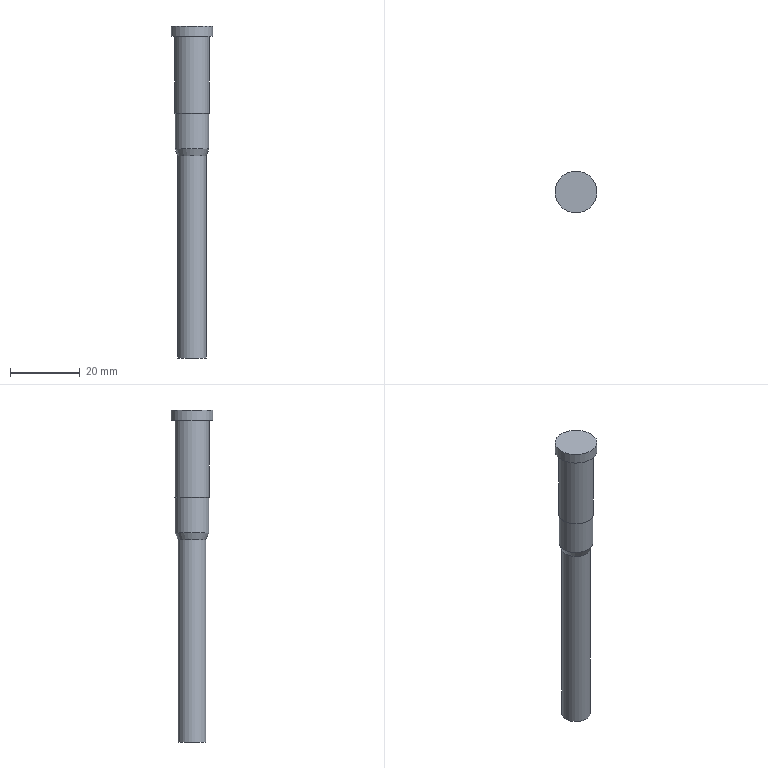Component | NX | PUNCH_2 | 1 solid | 9 faces | box 12 x 12 x 95 mm | volume 5896 mm3 | cylinder 4 | plane 3 | cone 2 | commonest cylinder face diameters 10 x1 9.717 x1 8.06 x1 12 x1
STEP:
#1=CARTESIAN_POINT('',(0.,0.,0.));
#2=DIRECTION('',(0.,0.,1.));
#3=DIRECTION('',(1.,0.,0.));
#4=AXIS2_PLACEMENT_3D('',#1,#2,#3);
#5=CARTESIAN_POINT('',(120.,0.,170.));
#6=VERTEX_POINT('',#5);
#7=CARTESIAN_POINT('',(125.,0.,170.));
#8=DIRECTION('',(0.,0.,-1.));
#9=DIRECTION('',(-1.,0.,0.));
#10=AXIS2_PLACEMENT_3D('',#7,#8,#9);
#11=CIRCLE('',#10,5.);
#12=CARTESIAN_POINT('',(125.,0.,195.));
#13=DIRECTION('',(0.,0.,-1.));
#14=DIRECTION('',(-1.,0.,0.));
#15=AXIS2_PLACEMENT_3D('',#12,#13,#14);
#16=CYLINDRICAL_SURFACE('',#15,5.);
#17=CARTESIAN_POINT('',(0.,25.));
#18=DIRECTION('',(1.,0.));
#19=VECTOR('',#18,1.);
#20=LINE('',#17,#19);
#21=(GEOMETRIC_REPRESENTATION_CONTEXT(2)PARAMETRIC_REPRESENTATION_CONTEXT()REPRESENTATION_CONTEXT('',''));
#22=DEFINITIONAL_REPRESENTATION('',(#20),#21);
#23=PCURVE('',#16,#22);
#24=CARTESIAN_POINT('',(125.,0.,170.));
#25=DIRECTION('',(0.,0.,1.));
#26=DIRECTION('',(1.,0.,0.));
#27=AXIS2_PLACEMENT_3D('',#24,#25,#26);
#28=CONICAL_SURFACE('',#27,5.,0.7854);
#29=CARTESIAN_POINT('',(9.425,0.));
#30=DIRECTION('',(-1.,0.));
#31=VECTOR('',#30,1.);
#32=LINE('',#29,#31);
#33=(GEOMETRIC_REPRESENTATION_CONTEXT(2)PARAMETRIC_REPRESENTATION_CONTEXT()REPRESENTATION_CONTEXT('',''));
#34=DEFINITIONAL_REPRESENTATION('',(#32),#33);
#35=PCURVE('',#28,#34);
#36=SURFACE_CURVE('',#11,(#23,#35),.PCURVE_S1.);
#37=EDGE_CURVE('',#6,#6,#36,.T.);
#38=ORIENTED_EDGE('',*,*,#37,.F.);
#39=CARTESIAN_POINT('',(120.,0.,192.));
#40=VERTEX_POINT('',#39);
#41=CARTESIAN_POINT('',(120.,-0.,192.));
#42=CARTESIAN_POINT('',(120.,-0.,170.));
#43=B_SPLINE_CURVE_WITH_KNOTS('',1,(#41,#42),.UNSPECIFIED.,.F.,.F.,(2,2),(3.,25.),.PIECEWISE_BEZIER_KNOTS.);
#44=CARTESIAN_POINT('',(0.,0.));
#45=DIRECTION('',(0.,1.));
#46=VECTOR('',#45,1.);
#47=LINE('',#44,#46);
#48=(GEOMETRIC_REPRESENTATION_CONTEXT(2)PARAMETRIC_REPRESENTATION_CONTEXT()REPRESENTATION_CONTEXT('',''));
#49=DEFINITIONAL_REPRESENTATION('',(#47),#48);
#50=PCURVE('',#16,#49);
#51=CARTESIAN_POINT('',(6.283,0.));
#52=DIRECTION('',(0.,1.));
#53=VECTOR('',#52,1.);
#54=LINE('',#51,#53);
#55=(GEOMETRIC_REPRESENTATION_CONTEXT(2)PARAMETRIC_REPRESENTATION_CONTEXT()REPRESENTATION_CONTEXT('',''));
#56=DEFINITIONAL_REPRESENTATION('',(#54),#55);
#57=PCURVE('',#16,#56);
#58=SEAM_CURVE('',#43,(#50,#57),.PCURVE_S1.);
#59=EDGE_CURVE('',#40,#6,#58,.T.);
#60=ORIENTED_EDGE('',*,*,#59,.F.);
#61=CARTESIAN_POINT('',(125.,0.,192.));
#62=DIRECTION('',(0.,0.,-1.));
#63=DIRECTION('',(-1.,0.,0.));
#64=AXIS2_PLACEMENT_3D('',#61,#62,#63);
#65=CIRCLE('',#64,5.);
#66=CARTESIAN_POINT('',(0.,3.));
#67=DIRECTION('',(1.,0.));
#68=VECTOR('',#67,1.);
#69=LINE('',#66,#68);
#70=(GEOMETRIC_REPRESENTATION_CONTEXT(2)PARAMETRIC_REPRESENTATION_CONTEXT()REPRESENTATION_CONTEXT('',''));
#71=DEFINITIONAL_REPRESENTATION('',(#69),#70);
#72=PCURVE('',#16,#71);
#73=CARTESIAN_POINT('',(131.,0.,192.));
#74=DIRECTION('',(0.,0.,1.));
#75=DIRECTION('',(1.,0.,0.));
#76=AXIS2_PLACEMENT_3D('',#73,#74,#75);
#77=PLANE('',#76);
#78=CARTESIAN_POINT('',(-11.,0.));
#79=CARTESIAN_POINT('',(-11.,8.66));
#80=CARTESIAN_POINT('',(-3.5,4.33));
#81=CARTESIAN_POINT('',(4.,0.));
#82=CARTESIAN_POINT('',(-3.5,-4.33));
#83=CARTESIAN_POINT('',(-11.,-8.66));
#84=CARTESIAN_POINT('',(-11.,0.));
#85=(BOUNDED_CURVE()B_SPLINE_CURVE(2,(#78,#79,#80,#81,#82,#83,#84),.UNSPECIFIED.,.T.,.F.)B_SPLINE_CURVE_WITH_KNOTS((1,2,2,2,2,1),(-2.094,0.,2.094,4.189,6.283,8.378),.UNSPECIFIED.)CURVE()GEOMETRIC_REPRESENTATION_ITEM()RATIONAL_B_SPLINE_CURVE((1.,0.5,1.,0.5,1.,0.5,1.))REPRESENTATION_ITEM(''));
#86=(GEOMETRIC_REPRESENTATION_CONTEXT(2)PARAMETRIC_REPRESENTATION_CONTEXT()REPRESENTATION_CONTEXT('',''));
#87=DEFINITIONAL_REPRESENTATION('',(#85),#86);
#88=PCURVE('',#77,#87);
#89=SURFACE_CURVE('',#65,(#72,#88),.PCURVE_S1.);
#90=EDGE_CURVE('',#40,#40,#89,.T.);
#91=ORIENTED_EDGE('',*,*,#90,.T.);
#92=ORIENTED_EDGE('',*,*,#59,.T.);
#93=EDGE_LOOP('',(#38,#60,#91,#92));
#94=FACE_BOUND('',#93,.T.);
#95=ADVANCED_FACE('',(#94),#16,.T.);
#96=CARTESIAN_POINT('',(120.141,0.,169.859));
#97=VERTEX_POINT('',#96);
#98=CARTESIAN_POINT('',(125.,0.,169.859));
#99=DIRECTION('',(0.,0.,-1.));
#100=DIRECTION('',(-1.,0.,0.));
#101=AXIS2_PLACEMENT_3D('',#98,#99,#100);
#102=CIRCLE('',#101,4.859);
#103=CARTESIAN_POINT('',(9.425,-0.1414));
#104=DIRECTION('',(-1.,0.));
#105=VECTOR('',#104,1.);
#106=LINE('',#103,#105);
#107=(GEOMETRIC_REPRESENTATION_CONTEXT(2)PARAMETRIC_REPRESENTATION_CONTEXT()REPRESENTATION_CONTEXT('',''));
#108=DEFINITIONAL_REPRESENTATION('',(#106),#107);
#109=PCURVE('',#28,#108);
#110=CARTESIAN_POINT('',(125.,0.,195.));
#111=DIRECTION('',(0.,0.,-1.));
#112=DIRECTION('',(-1.,0.,0.));
#113=AXIS2_PLACEMENT_3D('',#110,#111,#112);
#114=CYLINDRICAL_SURFACE('',#113,4.859);
#115=CARTESIAN_POINT('',(0.,25.141));
#116=DIRECTION('',(1.,0.));
#117=VECTOR('',#116,1.);
#118=LINE('',#115,#117);
#119=(GEOMETRIC_REPRESENTATION_CONTEXT(2)PARAMETRIC_REPRESENTATION_CONTEXT()REPRESENTATION_CONTEXT('',''));
#120=DEFINITIONAL_REPRESENTATION('',(#118),#119);
#121=PCURVE('',#114,#120);
#122=SURFACE_CURVE('',#102,(#109,#121),.PCURVE_S1.);
#123=EDGE_CURVE('',#97,#97,#122,.T.);
#124=ORIENTED_EDGE('',*,*,#123,.F.);
#125=CARTESIAN_POINT('',(120.141,0.,169.859));
#126=CARTESIAN_POINT('',(120.,0.,170.));
#127=B_SPLINE_CURVE_WITH_KNOTS('',1,(#125,#126),.UNSPECIFIED.,.F.,.F.,(2,2),(-0.2,0.),.PIECEWISE_BEZIER_KNOTS.);
#128=CARTESIAN_POINT('',(9.425,0.));
#129=DIRECTION('',(0.,1.));
#130=VECTOR('',#129,1.);
#131=LINE('',#128,#130);
#132=(GEOMETRIC_REPRESENTATION_CONTEXT(2)PARAMETRIC_REPRESENTATION_CONTEXT()REPRESENTATION_CONTEXT('',''));
#133=DEFINITIONAL_REPRESENTATION('',(#131),#132);
#134=PCURVE('',#28,#133);
#135=CARTESIAN_POINT('',(3.142,0.));
#136=DIRECTION('',(0.,1.));
#137=VECTOR('',#136,1.);
#138=LINE('',#135,#137);
#139=(GEOMETRIC_REPRESENTATION_CONTEXT(2)PARAMETRIC_REPRESENTATION_CONTEXT()REPRESENTATION_CONTEXT('',''));
#140=DEFINITIONAL_REPRESENTATION('',(#138),#139);
#141=PCURVE('',#28,#140);
#142=SEAM_CURVE('',#127,(#134,#141),.PCURVE_S1.);
#143=EDGE_CURVE('',#97,#6,#142,.T.);
#144=ORIENTED_EDGE('',*,*,#143,.T.);
#145=ORIENTED_EDGE('',*,*,#37,.T.);
#146=ORIENTED_EDGE('',*,*,#143,.F.);
#147=EDGE_LOOP('',(#124,#144,#145,#146));
#148=FACE_BOUND('',#147,.T.);
#149=ADVANCED_FACE('',(#148),#28,.T.);
#150=CARTESIAN_POINT('',(120.141,0.,159.859));
#151=VERTEX_POINT('',#150);
#152=CARTESIAN_POINT('',(125.,0.,159.859));
#153=DIRECTION('',(0.,0.,-1.));
#154=DIRECTION('',(-1.,0.,0.));
#155=AXIS2_PLACEMENT_3D('',#152,#153,#154);
#156=CIRCLE('',#155,4.859);
#157=CARTESIAN_POINT('',(0.,35.141));
#158=DIRECTION('',(1.,0.));
#159=VECTOR('',#158,1.);
#160=LINE('',#157,#159);
#161=(GEOMETRIC_REPRESENTATION_CONTEXT(2)PARAMETRIC_REPRESENTATION_CONTEXT()REPRESENTATION_CONTEXT('',''));
#162=DEFINITIONAL_REPRESENTATION('',(#160),#161);
#163=PCURVE('',#114,#162);
#164=CARTESIAN_POINT('',(125.,0.,159.859));
#165=DIRECTION('',(0.,0.,1.));
#166=DIRECTION('',(1.,0.,0.));
#167=AXIS2_PLACEMENT_3D('',#164,#165,#166);
#168=CONICAL_SURFACE('',#167,4.859,0.3928);
#169=CARTESIAN_POINT('',(9.425,0.));
#170=DIRECTION('',(-1.,0.));
#171=VECTOR('',#170,1.);
#172=LINE('',#169,#171);
#173=(GEOMETRIC_REPRESENTATION_CONTEXT(2)PARAMETRIC_REPRESENTATION_CONTEXT()REPRESENTATION_CONTEXT('',''));
#174=DEFINITIONAL_REPRESENTATION('',(#172),#173);
#175=PCURVE('',#168,#174);
#176=SURFACE_CURVE('',#156,(#163,#175),.PCURVE_S1.);
#177=EDGE_CURVE('',#151,#151,#176,.T.);
#178=ORIENTED_EDGE('',*,*,#177,.F.);
#179=CARTESIAN_POINT('',(120.141,-0.,169.859));
#180=CARTESIAN_POINT('',(120.141,-0.,159.859));
#181=B_SPLINE_CURVE_WITH_KNOTS('',1,(#179,#180),.UNSPECIFIED.,.F.,.F.,(2,2),(25.141,35.141),.PIECEWISE_BEZIER_KNOTS.);
#182=CARTESIAN_POINT('',(0.,0.));
#183=DIRECTION('',(0.,1.));
#184=VECTOR('',#183,1.);
#185=LINE('',#182,#184);
#186=(GEOMETRIC_REPRESENTATION_CONTEXT(2)PARAMETRIC_REPRESENTATION_CONTEXT()REPRESENTATION_CONTEXT('',''));
#187=DEFINITIONAL_REPRESENTATION('',(#185),#186);
#188=PCURVE('',#114,#187);
#189=CARTESIAN_POINT('',(6.283,0.));
#190=DIRECTION('',(0.,1.));
#191=VECTOR('',#190,1.);
#192=LINE('',#189,#191);
#193=(GEOMETRIC_REPRESENTATION_CONTEXT(2)PARAMETRIC_REPRESENTATION_CONTEXT()REPRESENTATION_CONTEXT('',''));
#194=DEFINITIONAL_REPRESENTATION('',(#192),#193);
#195=PCURVE('',#114,#194);
#196=SEAM_CURVE('',#181,(#188,#195),.PCURVE_S1.);
#197=EDGE_CURVE('',#97,#151,#196,.T.);
#198=ORIENTED_EDGE('',*,*,#197,.F.);
#199=ORIENTED_EDGE('',*,*,#123,.T.);
#200=ORIENTED_EDGE('',*,*,#197,.T.);
#201=EDGE_LOOP('',(#178,#198,#199,#200));
#202=FACE_BOUND('',#201,.T.);
#203=ADVANCED_FACE('',(#202),#114,.T.);
#204=CARTESIAN_POINT('',(120.97,0.,157.859));
#205=VERTEX_POINT('',#204);
#206=CARTESIAN_POINT('',(125.,0.,157.859));
#207=DIRECTION('',(0.,0.,-1.));
#208=DIRECTION('',(-1.,0.,0.));
#209=AXIS2_PLACEMENT_3D('',#206,#207,#208);
#210=CIRCLE('',#209,4.03);
#211=CARTESIAN_POINT('',(9.425,-2.));
#212=DIRECTION('',(-1.,0.));
#213=VECTOR('',#212,1.);
#214=LINE('',#211,#213);
#215=(GEOMETRIC_REPRESENTATION_CONTEXT(2)PARAMETRIC_REPRESENTATION_CONTEXT()REPRESENTATION_CONTEXT('',''));
#216=DEFINITIONAL_REPRESENTATION('',(#214),#215);
#217=PCURVE('',#168,#216);
#218=CARTESIAN_POINT('',(125.,0.,195.));
#219=DIRECTION('',(0.,0.,-1.));
#220=DIRECTION('',(-1.,0.,0.));
#221=AXIS2_PLACEMENT_3D('',#218,#219,#220);
#222=CYLINDRICAL_SURFACE('',#221,4.03);
#223=CARTESIAN_POINT('',(0.,37.141));
#224=DIRECTION('',(1.,0.));
#225=VECTOR('',#224,1.);
#226=LINE('',#223,#225);
#227=(GEOMETRIC_REPRESENTATION_CONTEXT(2)PARAMETRIC_REPRESENTATION_CONTEXT()REPRESENTATION_CONTEXT('',''));
#228=DEFINITIONAL_REPRESENTATION('',(#226),#227);
#229=PCURVE('',#222,#228);
#230=SURFACE_CURVE('',#210,(#217,#229),.PCURVE_S1.);
#231=EDGE_CURVE('',#205,#205,#230,.T.);
#232=ORIENTED_EDGE('',*,*,#231,.F.);
#233=CARTESIAN_POINT('',(120.97,0.,157.859));
#234=CARTESIAN_POINT('',(120.141,0.,159.859));
#235=B_SPLINE_CURVE_WITH_KNOTS('',1,(#233,#234),.UNSPECIFIED.,.F.,.F.,(2,2),(-2.165,0.),.PIECEWISE_BEZIER_KNOTS.);
#236=CARTESIAN_POINT('',(9.425,0.));
#237=DIRECTION('',(0.,1.));
#238=VECTOR('',#237,1.);
#239=LINE('',#236,#238);
#240=(GEOMETRIC_REPRESENTATION_CONTEXT(2)PARAMETRIC_REPRESENTATION_CONTEXT()REPRESENTATION_CONTEXT('',''));
#241=DEFINITIONAL_REPRESENTATION('',(#239),#240);
#242=PCURVE('',#168,#241);
#243=CARTESIAN_POINT('',(3.142,0.));
#244=DIRECTION('',(0.,1.));
#245=VECTOR('',#244,1.);
#246=LINE('',#243,#245);
#247=(GEOMETRIC_REPRESENTATION_CONTEXT(2)PARAMETRIC_REPRESENTATION_CONTEXT()REPRESENTATION_CONTEXT('',''));
#248=DEFINITIONAL_REPRESENTATION('',(#246),#247);
#249=PCURVE('',#168,#248);
#250=SEAM_CURVE('',#235,(#242,#249),.PCURVE_S1.);
#251=EDGE_CURVE('',#205,#151,#250,.T.);
#252=ORIENTED_EDGE('',*,*,#251,.T.);
#253=ORIENTED_EDGE('',*,*,#177,.T.);
#254=ORIENTED_EDGE('',*,*,#251,.F.);
#255=EDGE_LOOP('',(#232,#252,#253,#254));
#256=FACE_BOUND('',#255,.T.);
#257=ADVANCED_FACE('',(#256),#168,.T.);
#258=CARTESIAN_POINT('',(120.97,0.,100.));
#259=VERTEX_POINT('',#258);
#260=CARTESIAN_POINT('',(125.,0.,100.));
#261=DIRECTION('',(0.,0.,-1.));
#262=DIRECTION('',(-1.,0.,0.));
#263=AXIS2_PLACEMENT_3D('',#260,#261,#262);
#264=CIRCLE('',#263,4.03);
#265=CARTESIAN_POINT('',(0.,95.));
#266=DIRECTION('',(1.,0.));
#267=VECTOR('',#266,1.);
#268=LINE('',#265,#267);
#269=(GEOMETRIC_REPRESENTATION_CONTEXT(2)PARAMETRIC_REPRESENTATION_CONTEXT()REPRESENTATION_CONTEXT('',''));
#270=DEFINITIONAL_REPRESENTATION('',(#268),#269);
#271=PCURVE('',#222,#270);
#272=CARTESIAN_POINT('',(129.03,0.,100.));
#273=DIRECTION('',(0.,0.,1.));
#274=DIRECTION('',(1.,0.,0.));
#275=AXIS2_PLACEMENT_3D('',#272,#273,#274);
#276=PLANE('',#275);
#277=CARTESIAN_POINT('',(-8.06,0.));
#278=CARTESIAN_POINT('',(-8.06,6.98));
#279=CARTESIAN_POINT('',(-2.015,3.49));
#280=CARTESIAN_POINT('',(4.03,0.));
#281=CARTESIAN_POINT('',(-2.015,-3.49));
#282=CARTESIAN_POINT('',(-8.06,-6.98));
#283=CARTESIAN_POINT('',(-8.06,0.));
#284=(BOUNDED_CURVE()B_SPLINE_CURVE(2,(#277,#278,#279,#280,#281,#282,#283),.UNSPECIFIED.,.T.,.F.)B_SPLINE_CURVE_WITH_KNOTS((1,2,2,2,2,1),(-2.094,0.,2.094,4.189,6.283,8.378),.UNSPECIFIED.)CURVE()GEOMETRIC_REPRESENTATION_ITEM()RATIONAL_B_SPLINE_CURVE((1.,0.5,1.,0.5,1.,0.5,1.))REPRESENTATION_ITEM(''));
#285=(GEOMETRIC_REPRESENTATION_CONTEXT(2)PARAMETRIC_REPRESENTATION_CONTEXT()REPRESENTATION_CONTEXT('',''));
#286=DEFINITIONAL_REPRESENTATION('',(#284),#285);
#287=PCURVE('',#276,#286);
#288=SURFACE_CURVE('',#264,(#271,#287),.PCURVE_S1.);
#289=EDGE_CURVE('',#259,#259,#288,.T.);
#290=ORIENTED_EDGE('',*,*,#289,.F.);
#291=CARTESIAN_POINT('',(120.97,-0.,157.859));
#292=CARTESIAN_POINT('',(120.97,-0.,100.));
#293=B_SPLINE_CURVE_WITH_KNOTS('',1,(#291,#292),.UNSPECIFIED.,.F.,.F.,(2,2),(37.141,95.),.PIECEWISE_BEZIER_KNOTS.);
#294=CARTESIAN_POINT('',(0.,0.));
#295=DIRECTION('',(0.,1.));
#296=VECTOR('',#295,1.);
#297=LINE('',#294,#296);
#298=(GEOMETRIC_REPRESENTATION_CONTEXT(2)PARAMETRIC_REPRESENTATION_CONTEXT()REPRESENTATION_CONTEXT('',''));
#299=DEFINITIONAL_REPRESENTATION('',(#297),#298);
#300=PCURVE('',#222,#299);
#301=CARTESIAN_POINT('',(6.283,0.));
#302=DIRECTION('',(0.,1.));
#303=VECTOR('',#302,1.);
#304=LINE('',#301,#303);
#305=(GEOMETRIC_REPRESENTATION_CONTEXT(2)PARAMETRIC_REPRESENTATION_CONTEXT()REPRESENTATION_CONTEXT('',''));
#306=DEFINITIONAL_REPRESENTATION('',(#304),#305);
#307=PCURVE('',#222,#306);
#308=SEAM_CURVE('',#293,(#300,#307),.PCURVE_S1.);
#309=EDGE_CURVE('',#205,#259,#308,.T.);
#310=ORIENTED_EDGE('',*,*,#309,.F.);
#311=ORIENTED_EDGE('',*,*,#231,.T.);
#312=ORIENTED_EDGE('',*,*,#309,.T.);
#313=EDGE_LOOP('',(#290,#310,#311,#312));
#314=FACE_BOUND('',#313,.T.);
#315=ADVANCED_FACE('',(#314),#222,.T.);
#316=ORIENTED_EDGE('',*,*,#289,.T.);
#317=EDGE_LOOP('',(#316));
#318=FACE_BOUND('',#317,.T.);
#319=ADVANCED_FACE('',(#318),#276,.F.);
#320=CARTESIAN_POINT('',(119.,0.,195.));
#321=VERTEX_POINT('',#320);
#322=CARTESIAN_POINT('',(125.,0.,195.));
#323=DIRECTION('',(0.,0.,-1.));
#324=DIRECTION('',(-1.,0.,0.));
#325=AXIS2_PLACEMENT_3D('',#322,#323,#324);
#326=CIRCLE('',#325,6.);
#327=CARTESIAN_POINT('',(125.,0.,195.));
#328=DIRECTION('',(0.,0.,-1.));
#329=DIRECTION('',(-1.,0.,0.));
#330=AXIS2_PLACEMENT_3D('',#327,#328,#329);
#331=PLANE('',#330);
#332=CARTESIAN_POINT('',(0.,0.));
#333=DIRECTION('',(1.,0.));
#334=AXIS2_PLACEMENT_2D('',#332,#333);
#335=CIRCLE('',#334,6.);
#336=(GEOMETRIC_REPRESENTATION_CONTEXT(2)PARAMETRIC_REPRESENTATION_CONTEXT()REPRESENTATION_CONTEXT('',''));
#337=DEFINITIONAL_REPRESENTATION('',(#335),#336);
#338=PCURVE('',#331,#337);
#339=CARTESIAN_POINT('',(125.,0.,195.));
#340=DIRECTION('',(0.,0.,-1.));
#341=DIRECTION('',(-1.,0.,0.));
#342=AXIS2_PLACEMENT_3D('',#339,#340,#341);
#343=CYLINDRICAL_SURFACE('',#342,6.);
#344=CARTESIAN_POINT('',(0.,0.));
#345=DIRECTION('',(1.,0.));
#346=VECTOR('',#345,1.);
#347=LINE('',#344,#346);
#348=(GEOMETRIC_REPRESENTATION_CONTEXT(2)PARAMETRIC_REPRESENTATION_CONTEXT()REPRESENTATION_CONTEXT('',''));
#349=DEFINITIONAL_REPRESENTATION('',(#347),#348);
#350=PCURVE('',#343,#349);
#351=SURFACE_CURVE('',#326,(#338,#350),.PCURVE_S1.);
#352=EDGE_CURVE('',#321,#321,#351,.T.);
#353=ORIENTED_EDGE('',*,*,#352,.F.);
#354=EDGE_LOOP('',(#353));
#355=FACE_BOUND('',#354,.T.);
#356=ADVANCED_FACE('',(#355),#331,.F.);
#357=CARTESIAN_POINT('',(119.,0.,192.));
#358=VERTEX_POINT('',#357);
#359=CARTESIAN_POINT('',(125.,0.,192.));
#360=DIRECTION('',(0.,0.,-1.));
#361=DIRECTION('',(-1.,0.,0.));
#362=AXIS2_PLACEMENT_3D('',#359,#360,#361);
#363=CIRCLE('',#362,6.);
#364=CARTESIAN_POINT('',(0.,3.));
#365=DIRECTION('',(1.,0.));
#366=VECTOR('',#365,1.);
#367=LINE('',#364,#366);
#368=(GEOMETRIC_REPRESENTATION_CONTEXT(2)PARAMETRIC_REPRESENTATION_CONTEXT()REPRESENTATION_CONTEXT('',''));
#369=DEFINITIONAL_REPRESENTATION('',(#367),#368);
#370=PCURVE('',#343,#369);
#371=CARTESIAN_POINT('',(-12.,0.));
#372=CARTESIAN_POINT('',(-12.,10.392));
#373=CARTESIAN_POINT('',(-3.,5.196));
#374=CARTESIAN_POINT('',(6.,0.));
#375=CARTESIAN_POINT('',(-3.,-5.196));
#376=CARTESIAN_POINT('',(-12.,-10.392));
#377=CARTESIAN_POINT('',(-12.,0.));
#378=(BOUNDED_CURVE()B_SPLINE_CURVE(2,(#371,#372,#373,#374,#375,#376,#377),.UNSPECIFIED.,.T.,.F.)B_SPLINE_CURVE_WITH_KNOTS((1,2,2,2,2,1),(-2.094,0.,2.094,4.189,6.283,8.378),.UNSPECIFIED.)CURVE()GEOMETRIC_REPRESENTATION_ITEM()RATIONAL_B_SPLINE_CURVE((1.,0.5,1.,0.5,1.,0.5,1.))REPRESENTATION_ITEM(''));
#379=(GEOMETRIC_REPRESENTATION_CONTEXT(2)PARAMETRIC_REPRESENTATION_CONTEXT()REPRESENTATION_CONTEXT('',''));
#380=DEFINITIONAL_REPRESENTATION('',(#378),#379);
#381=PCURVE('',#77,#380);
#382=SURFACE_CURVE('',#363,(#370,#381),.PCURVE_S1.);
#383=EDGE_CURVE('',#358,#358,#382,.T.);
#384=ORIENTED_EDGE('',*,*,#383,.F.);
#385=CARTESIAN_POINT('',(119.,-0.,195.));
#386=CARTESIAN_POINT('',(119.,-0.,192.));
#387=B_SPLINE_CURVE_WITH_KNOTS('',1,(#385,#386),.UNSPECIFIED.,.F.,.F.,(2,2),(0.,3.),.PIECEWISE_BEZIER_KNOTS.);
#388=CARTESIAN_POINT('',(0.,0.));
#389=DIRECTION('',(0.,1.));
#390=VECTOR('',#389,1.);
#391=LINE('',#388,#390);
#392=(GEOMETRIC_REPRESENTATION_CONTEXT(2)PARAMETRIC_REPRESENTATION_CONTEXT()REPRESENTATION_CONTEXT('',''));
#393=DEFINITIONAL_REPRESENTATION('',(#391),#392);
#394=PCURVE('',#343,#393);
#395=CARTESIAN_POINT('',(6.283,0.));
#396=DIRECTION('',(0.,1.));
#397=VECTOR('',#396,1.);
#398=LINE('',#395,#397);
#399=(GEOMETRIC_REPRESENTATION_CONTEXT(2)PARAMETRIC_REPRESENTATION_CONTEXT()REPRESENTATION_CONTEXT('',''));
#400=DEFINITIONAL_REPRESENTATION('',(#398),#399);
#401=PCURVE('',#343,#400);
#402=SEAM_CURVE('',#387,(#394,#401),.PCURVE_S1.);
#403=EDGE_CURVE('',#321,#358,#402,.T.);
#404=ORIENTED_EDGE('',*,*,#403,.F.);
#405=ORIENTED_EDGE('',*,*,#352,.T.);
#406=ORIENTED_EDGE('',*,*,#403,.T.);
#407=EDGE_LOOP('',(#384,#404,#405,#406));
#408=FACE_BOUND('',#407,.T.);
#409=ADVANCED_FACE('',(#408),#343,.T.);
#410=ORIENTED_EDGE('',*,*,#90,.F.);
#411=EDGE_LOOP('',(#410));
#412=FACE_BOUND('',#411,.T.);
#413=ORIENTED_EDGE('',*,*,#383,.T.);
#414=EDGE_LOOP('',(#413));
#415=FACE_BOUND('',#414,.T.);
#416=ADVANCED_FACE('',(#412,#415),#77,.F.);
#417=CLOSED_SHELL('',(#95,#149,#203,#257,#315,#319,#356,#409,#416));
#418=MANIFOLD_SOLID_BREP('',#417);
#419=(LENGTH_UNIT()NAMED_UNIT(*)SI_UNIT(.MILLI.,.METRE.));
#420=UNCERTAINTY_MEASURE_WITH_UNIT(LENGTH_MEASURE(0.00001),#419,'','');
#421=(NAMED_UNIT(*)PLANE_ANGLE_UNIT()SI_UNIT($,.RADIAN.));
#422=(NAMED_UNIT(*)SI_UNIT($,.STERADIAN.)SOLID_ANGLE_UNIT());
#423=(GEOMETRIC_REPRESENTATION_CONTEXT(3)GLOBAL_UNCERTAINTY_ASSIGNED_CONTEXT((#420))GLOBAL_UNIT_ASSIGNED_CONTEXT((#419,#421,#422))REPRESENTATION_CONTEXT('',''));
#424=ADVANCED_BREP_SHAPE_REPRESENTATION('',(#4,#418),#423);